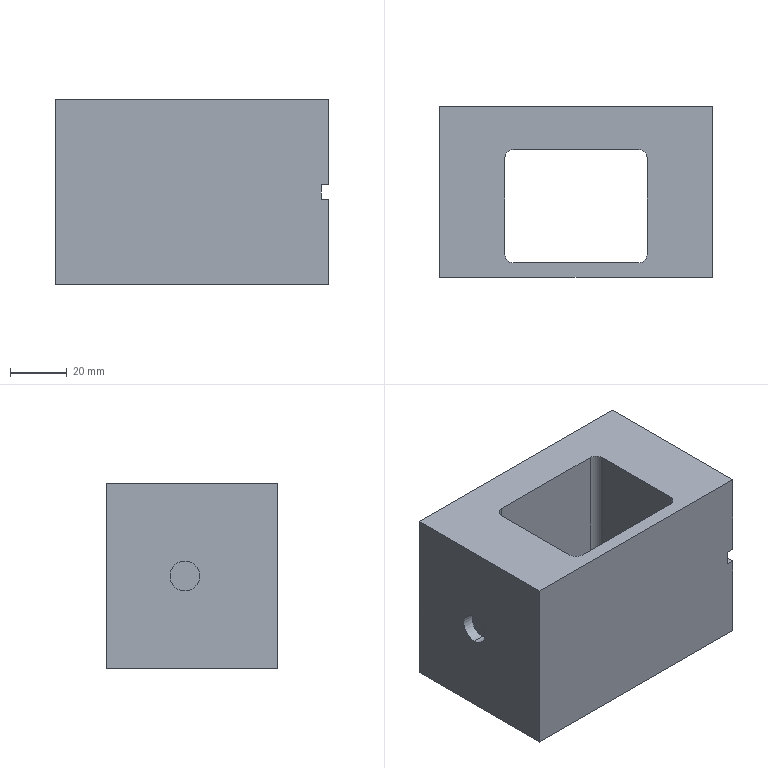Component | SolidWorks | CuttingDie-1_-Mold01-2-1 | 1 solid | 21 faces | box 96 x 60 x 65 mm | volume 243806 mm3 | plane 15 | cylinder 6 | commonest cylinder face diameters 6 x4 10.5 x2
build123d program:
from build123d import *

# Parameters (mm, degrees)
SKETCH1_W           = 65
SKETCH1_H           = 96
BOSS_EXTRUDE1_DEPTH = 32.5
SKETCH3_W           = 5
SKETCH3_H           = 2.5
CUT_EXTRUDE2_DEPTH  = 88.093
SKETCH4_R           = 5.25
CUT_EXTRUDE3_DEPTH  = 4
SKETCH6_W           = 65
SKETCH6_H           = 5
CUT_EXTRUDE5_DEPTH  = 107.435
CUT_EXTRUDE7_DEPTH  = 88.093


with BuildPart() as part:
    # Sketch1 → Boss-Extrude1 (new, symmetric)
    with BuildSketch(Plane(origin=(0, 0, 0), x_dir=(1, 0, 0), z_dir=(0, 1, 0))):
        Rectangle(SKETCH1_W, SKETCH1_H)
    extrude(amount=BOSS_EXTRUDE1_DEPTH, both=True)

    # Sketch3 → Cut-Extrude2 (cut, through all)
    with BuildSketch(Plane(origin=(0, 32.5, 0), x_dir=(1, 0, 0), z_dir=(0, 1, 0))):
        with Locations((0, 46.75)):
            Rectangle(SKETCH3_W, SKETCH3_H)
    extrude(amount=-CUT_EXTRUDE2_DEPTH, mode=Mode.SUBTRACT)

    # Sketch4 → Cut-Extrude3 (cut)
    with BuildSketch(Plane.XY.offset(48)):
        Circle(SKETCH4_R)
    extrude(amount=-CUT_EXTRUDE3_DEPTH, mode=Mode.SUBTRACT)

    # Sketch6 → Cut-Extrude5 (cut, through all)
    with BuildSketch(Plane.XY.offset(48)):
        with Locations((0, 30)):
            Rectangle(SKETCH6_W, SKETCH6_H)
    extrude(amount=-CUT_EXTRUDE5_DEPTH, mode=Mode.SUBTRACT)

    # Sketch2 → Cut-Extrude7 (cut, through all)
    with BuildSketch(Plane(origin=(32.5, 0, 0), x_dir=(0, 0, -1), z_dir=(1, 0, 0))):
        with BuildLine():
            Line((-22, -27.5), (22, -27.5))
            ThreePointArc((22, -27.5), (24.121, -26.621), (25, -24.5))
            Line((25, -24.5), (25, 9.5))
            ThreePointArc((25, 9.5), (24.121, 11.621), (22, 12.5))
            Line((22, 12.5), (-22, 12.5))
            ThreePointArc((-22, 12.5), (-24.121, 11.621), (-25, 9.5))
            Line((-25, 9.5), (-25, -24.5))
            ThreePointArc((-25, -24.5), (-24.121, -26.621), (-22, -27.5))
        make_face()
    extrude(amount=-CUT_EXTRUDE7_DEPTH, mode=Mode.SUBTRACT)


solid = part.part

# Placed as in the assembly
solid = solid.moved(Location((-439.272, -274.266, 1034.5), (0, -90, 0)))
STEP:
#1=COLOUR_RGB('',0.7922,0.8196,0.9333);
#2=FILL_AREA_STYLE_COLOUR('',#1);
#3=FILL_AREA_STYLE('',(#2));
#4=SURFACE_STYLE_FILL_AREA(#3);
#5=SURFACE_SIDE_STYLE('',(#4));
#6=SURFACE_STYLE_USAGE(.BOTH.,#5);
#7=PRESENTATION_STYLE_ASSIGNMENT((#6));
#8=CARTESIAN_POINT('',(-19.026,-10.798,40.522));
#9=VERTEX_POINT('',#8);
#10=CARTESIAN_POINT('',(-19.026,-10.798,40.935));
#11=VERTEX_POINT('',#10);
#12=CARTESIAN_POINT('',(-19.026,-10.798,40.728));
#13=DIRECTION('',(-1.,-0.,-0.));
#14=DIRECTION('',(0.,0.,1.));
#15=AXIS2_PLACEMENT_3D('',#12,#13,#14);
#16=CIRCLE('',#15,0.2067);
#17=EDGE_CURVE('',#9,#11,#16,.T.);
#18=ORIENTED_EDGE('',*,*,#17,.F.);
#19=CARTESIAN_POINT('',(-19.184,-10.798,40.522));
#20=VERTEX_POINT('',#19);
#21=CARTESIAN_POINT('',(-19.026,-10.798,40.522));
#22=DIRECTION('',(-1.,-0.,-0.));
#23=VECTOR('',#22,39.37);
#24=LINE('',#21,#23);
#25=EDGE_CURVE('',#9,#20,#24,.T.);
#26=ORIENTED_EDGE('',*,*,#25,.T.);
#27=CARTESIAN_POINT('',(-19.184,-10.798,40.935));
#28=VERTEX_POINT('',#27);
#29=CARTESIAN_POINT('',(-19.184,-10.798,40.728));
#30=DIRECTION('',(-1.,-0.,-0.));
#31=DIRECTION('',(0.,0.,1.));
#32=AXIS2_PLACEMENT_3D('',#29,#30,#31);
#33=CIRCLE('',#32,0.2067);
#34=EDGE_CURVE('',#20,#28,#33,.T.);
#35=ORIENTED_EDGE('',*,*,#34,.T.);
#36=CARTESIAN_POINT('',(-19.026,-10.798,40.935));
#37=DIRECTION('',(-1.,-0.,-0.));
#38=VECTOR('',#37,39.37);
#39=LINE('',#36,#38);
#40=EDGE_CURVE('',#11,#28,#39,.T.);
#41=ORIENTED_EDGE('',*,*,#40,.F.);
#42=EDGE_LOOP('',(#18,#26,#35,#41));
#43=FACE_OUTER_BOUND('',#42,.T.);
#44=CARTESIAN_POINT('',(-19.026,-10.798,40.728));
#45=DIRECTION('',(-1.,-0.,-0.));
#46=DIRECTION('',(0.,0.,1.));
#47=AXIS2_PLACEMENT_3D('',#44,#45,#46);
#48=CYLINDRICAL_SURFACE('',#47,0.2067);
#49=ADVANCED_FACE('',(#43),#48,.F.);
#50=CARTESIAN_POINT('',(-15.404,-9.715,39.449));
#51=VERTEX_POINT('',#50);
#52=CARTESIAN_POINT('',(-15.404,-12.077,39.449));
#53=VERTEX_POINT('',#52);
#54=CARTESIAN_POINT('',(-15.404,-9.518,39.449));
#55=DIRECTION('',(0.,-1.,-0.));
#56=VECTOR('',#55,39.37);
#57=LINE('',#54,#56);
#58=EDGE_CURVE('',#51,#53,#57,.T.);
#59=ORIENTED_EDGE('',*,*,#58,.F.);
#60=CARTESIAN_POINT('',(-15.404,-9.715,40.63));
#61=VERTEX_POINT('',#60);
#62=CARTESIAN_POINT('',(-15.404,-9.715,39.449));
#63=DIRECTION('',(-0.,-0.,1.));
#64=VECTOR('',#63,39.37);
#65=LINE('',#62,#64);
#66=EDGE_CURVE('',#51,#61,#65,.T.);
#67=ORIENTED_EDGE('',*,*,#66,.T.);
#68=CARTESIAN_POINT('',(-15.404,-12.077,40.63));
#69=VERTEX_POINT('',#68);
#70=CARTESIAN_POINT('',(-15.404,-12.077,40.63));
#71=DIRECTION('',(-0.,1.,0.));
#72=VECTOR('',#71,39.37);
#73=LINE('',#70,#72);
#74=EDGE_CURVE('',#69,#61,#73,.T.);
#75=ORIENTED_EDGE('',*,*,#74,.F.);
#76=CARTESIAN_POINT('',(-15.404,-12.077,39.449));
#77=DIRECTION('',(0.,0.,-1.));
#78=VECTOR('',#77,39.37);
#79=LINE('',#76,#78);
#80=EDGE_CURVE('',#69,#53,#79,.T.);
#81=ORIENTED_EDGE('',*,*,#80,.T.);
#82=EDGE_LOOP('',(#59,#67,#75,#81));
#83=FACE_OUTER_BOUND('',#82,.T.);
#84=CARTESIAN_POINT('',(-15.404,-9.518,39.449));
#85=DIRECTION('',(-1.,-0.,-0.));
#86=DIRECTION('',(-0.,-0.,1.));
#87=AXIS2_PLACEMENT_3D('',#84,#85,#86);
#88=PLANE('',#87);
#89=ADVANCED_FACE('',(#83),#88,.F.);
#90=CARTESIAN_POINT('',(-16.31,-11.762,42.008));
#91=VERTEX_POINT('',#90);
#92=CARTESIAN_POINT('',(-16.31,-10.424,42.008));
#93=VERTEX_POINT('',#92);
#94=CARTESIAN_POINT('',(-16.31,-11.762,42.008));
#95=DIRECTION('',(-0.,1.,0.));
#96=VECTOR('',#95,39.37);
#97=LINE('',#94,#96);
#98=EDGE_CURVE('',#91,#93,#97,.T.);
#99=ORIENTED_EDGE('',*,*,#98,.F.);
#100=CARTESIAN_POINT('',(-16.428,-11.881,42.008));
#101=VERTEX_POINT('',#100);
#102=CARTESIAN_POINT('',(-16.428,-11.762,42.008));
#103=DIRECTION('',(-0.,-0.,1.));
#104=DIRECTION('',(1.,0.,0.));
#105=AXIS2_PLACEMENT_3D('',#102,#103,#104);
#106=CIRCLE('',#105,0.1181);
#107=EDGE_CURVE('',#101,#91,#106,.T.);
#108=ORIENTED_EDGE('',*,*,#107,.F.);
#109=CARTESIAN_POINT('',(-18.16,-11.881,42.008));
#110=VERTEX_POINT('',#109);
#111=CARTESIAN_POINT('',(-18.16,-11.881,42.008));
#112=DIRECTION('',(1.,0.,0.));
#113=VECTOR('',#112,39.37);
#114=LINE('',#111,#113);
#115=EDGE_CURVE('',#110,#101,#114,.T.);
#116=ORIENTED_EDGE('',*,*,#115,.F.);
#117=CARTESIAN_POINT('',(-18.278,-11.762,42.008));
#118=VERTEX_POINT('',#117);
#119=CARTESIAN_POINT('',(-18.16,-11.762,42.008));
#120=DIRECTION('',(-0.,-0.,1.));
#121=DIRECTION('',(-1.,0.,0.));
#122=AXIS2_PLACEMENT_3D('',#119,#120,#121);
#123=CIRCLE('',#122,0.1181);
#124=EDGE_CURVE('',#118,#110,#123,.T.);
#125=ORIENTED_EDGE('',*,*,#124,.F.);
#126=CARTESIAN_POINT('',(-18.278,-10.424,42.008));
#127=VERTEX_POINT('',#126);
#128=CARTESIAN_POINT('',(-18.278,-11.762,42.008));
#129=DIRECTION('',(0.,-1.,-0.));
#130=VECTOR('',#129,39.37);
#131=LINE('',#128,#130);
#132=EDGE_CURVE('',#127,#118,#131,.T.);
#133=ORIENTED_EDGE('',*,*,#132,.F.);
#134=CARTESIAN_POINT('',(-18.16,-10.306,42.008));
#135=VERTEX_POINT('',#134);
#136=CARTESIAN_POINT('',(-18.16,-10.424,42.008));
#137=DIRECTION('',(-0.,-0.,1.));
#138=DIRECTION('',(-1.,0.,0.));
#139=AXIS2_PLACEMENT_3D('',#136,#137,#138);
#140=CIRCLE('',#139,0.1181);
#141=EDGE_CURVE('',#135,#127,#140,.T.);
#142=ORIENTED_EDGE('',*,*,#141,.F.);
#143=CARTESIAN_POINT('',(-16.428,-10.306,42.008));
#144=VERTEX_POINT('',#143);
#145=CARTESIAN_POINT('',(-18.16,-10.306,42.008));
#146=DIRECTION('',(-1.,-0.,-0.));
#147=VECTOR('',#146,39.37);
#148=LINE('',#145,#147);
#149=EDGE_CURVE('',#144,#135,#148,.T.);
#150=ORIENTED_EDGE('',*,*,#149,.F.);
#151=CARTESIAN_POINT('',(-16.428,-10.424,42.008));
#152=DIRECTION('',(-0.,-0.,1.));
#153=DIRECTION('',(-1.,0.,0.));
#154=AXIS2_PLACEMENT_3D('',#151,#152,#153);
#155=CIRCLE('',#154,0.1181);
#156=EDGE_CURVE('',#93,#144,#155,.T.);
#157=ORIENTED_EDGE('',*,*,#156,.F.);
#158=EDGE_LOOP('',(#99,#108,#116,#125,#133,#142,#150,#157));
#159=FACE_BOUND('',#158,.T.);
#160=CARTESIAN_POINT('',(-15.404,-9.715,42.008));
#161=VERTEX_POINT('',#160);
#162=CARTESIAN_POINT('',(-15.404,-12.077,42.008));
#163=VERTEX_POINT('',#162);
#164=CARTESIAN_POINT('',(-15.404,-9.518,42.008));
#165=DIRECTION('',(0.,-1.,-0.));
#166=VECTOR('',#165,39.37);
#167=LINE('',#164,#166);
#168=EDGE_CURVE('',#161,#163,#167,.T.);
#169=ORIENTED_EDGE('',*,*,#168,.F.);
#170=CARTESIAN_POINT('',(-19.184,-9.715,42.008));
#171=VERTEX_POINT('',#170);
#172=CARTESIAN_POINT('',(-15.404,-9.715,42.008));
#173=DIRECTION('',(-1.,-0.,-0.));
#174=VECTOR('',#173,39.37);
#175=LINE('',#172,#174);
#176=EDGE_CURVE('',#161,#171,#175,.T.);
#177=ORIENTED_EDGE('',*,*,#176,.T.);
#178=CARTESIAN_POINT('',(-19.184,-12.077,42.008));
#179=VERTEX_POINT('',#178);
#180=CARTESIAN_POINT('',(-19.184,-9.518,42.008));
#181=DIRECTION('',(0.,-1.,-0.));
#182=VECTOR('',#181,39.37);
#183=LINE('',#180,#182);
#184=EDGE_CURVE('',#171,#179,#183,.T.);
#185=ORIENTED_EDGE('',*,*,#184,.T.);
#186=CARTESIAN_POINT('',(-19.184,-12.077,42.008));
#187=DIRECTION('',(1.,0.,0.));
#188=VECTOR('',#187,39.37);
#189=LINE('',#186,#188);
#190=EDGE_CURVE('',#179,#163,#189,.T.);
#191=ORIENTED_EDGE('',*,*,#190,.T.);
#192=EDGE_LOOP('',(#169,#177,#185,#191));
#193=FACE_OUTER_BOUND('',#192,.T.);
#194=CARTESIAN_POINT('',(-19.184,-9.518,42.008));
#195=DIRECTION('',(0.,0.,-1.));
#196=DIRECTION('',(-1.,-0.,-0.));
#197=AXIS2_PLACEMENT_3D('',#194,#195,#196);
#198=PLANE('',#197);
#199=ADVANCED_FACE('',(#159,#193),#198,.F.);
#200=CARTESIAN_POINT('',(-15.404,-12.077,40.827));
#201=VERTEX_POINT('',#200);
#202=CARTESIAN_POINT('',(-15.404,-9.715,40.827));
#203=VERTEX_POINT('',#202);
#204=CARTESIAN_POINT('',(-15.404,-12.077,40.827));
#205=DIRECTION('',(-0.,1.,0.));
#206=VECTOR('',#205,39.37);
#207=LINE('',#204,#206);
#208=EDGE_CURVE('',#201,#203,#207,.T.);
#209=ORIENTED_EDGE('',*,*,#208,.T.);
#210=CARTESIAN_POINT('',(-15.404,-9.715,39.449));
#211=DIRECTION('',(-0.,-0.,1.));
#212=VECTOR('',#211,39.37);
#213=LINE('',#210,#212);
#214=EDGE_CURVE('',#203,#161,#213,.T.);
#215=ORIENTED_EDGE('',*,*,#214,.T.);
#216=ORIENTED_EDGE('',*,*,#168,.T.);
#217=CARTESIAN_POINT('',(-15.404,-12.077,39.449));
#218=DIRECTION('',(0.,0.,-1.));
#219=VECTOR('',#218,39.37);
#220=LINE('',#217,#219);
#221=EDGE_CURVE('',#163,#201,#220,.T.);
#222=ORIENTED_EDGE('',*,*,#221,.T.);
#223=EDGE_LOOP('',(#209,#215,#216,#222));
#224=FACE_OUTER_BOUND('',#223,.T.);
#225=CARTESIAN_POINT('',(-15.404,-9.518,39.449));
#226=DIRECTION('',(-1.,-0.,-0.));
#227=DIRECTION('',(-0.,-0.,1.));
#228=AXIS2_PLACEMENT_3D('',#225,#226,#227);
#229=PLANE('',#228);
#230=ADVANCED_FACE('',(#224),#229,.F.);
#231=CARTESIAN_POINT('',(-18.16,-11.881,39.449));
#232=VERTEX_POINT('',#231);
#233=CARTESIAN_POINT('',(-16.428,-11.881,39.449));
#234=VERTEX_POINT('',#233);
#235=CARTESIAN_POINT('',(-18.16,-11.881,39.449));
#236=DIRECTION('',(1.,0.,0.));
#237=VECTOR('',#236,39.37);
#238=LINE('',#235,#237);
#239=EDGE_CURVE('',#232,#234,#238,.T.);
#240=ORIENTED_EDGE('',*,*,#239,.T.);
#241=CARTESIAN_POINT('',(-16.31,-11.762,39.449));
#242=VERTEX_POINT('',#241);
#243=CARTESIAN_POINT('',(-16.428,-11.762,39.449));
#244=DIRECTION('',(-0.,-0.,1.));
#245=DIRECTION('',(1.,0.,0.));
#246=AXIS2_PLACEMENT_3D('',#243,#244,#245);
#247=CIRCLE('',#246,0.1181);
#248=EDGE_CURVE('',#234,#242,#247,.T.);
#249=ORIENTED_EDGE('',*,*,#248,.T.);
#250=CARTESIAN_POINT('',(-16.31,-10.424,39.449));
#251=VERTEX_POINT('',#250);
#252=CARTESIAN_POINT('',(-16.31,-11.762,39.449));
#253=DIRECTION('',(-0.,1.,0.));
#254=VECTOR('',#253,39.37);
#255=LINE('',#252,#254);
#256=EDGE_CURVE('',#242,#251,#255,.T.);
#257=ORIENTED_EDGE('',*,*,#256,.T.);
#258=CARTESIAN_POINT('',(-16.428,-10.306,39.449));
#259=VERTEX_POINT('',#258);
#260=CARTESIAN_POINT('',(-16.428,-10.424,39.449));
#261=DIRECTION('',(-0.,-0.,1.));
#262=DIRECTION('',(-1.,0.,0.));
#263=AXIS2_PLACEMENT_3D('',#260,#261,#262);
#264=CIRCLE('',#263,0.1181);
#265=EDGE_CURVE('',#251,#259,#264,.T.);
#266=ORIENTED_EDGE('',*,*,#265,.T.);
#267=CARTESIAN_POINT('',(-18.16,-10.306,39.449));
#268=VERTEX_POINT('',#267);
#269=CARTESIAN_POINT('',(-18.16,-10.306,39.449));
#270=DIRECTION('',(-1.,-0.,-0.));
#271=VECTOR('',#270,39.37);
#272=LINE('',#269,#271);
#273=EDGE_CURVE('',#259,#268,#272,.T.);
#274=ORIENTED_EDGE('',*,*,#273,.T.);
#275=CARTESIAN_POINT('',(-18.278,-10.424,39.449));
#276=VERTEX_POINT('',#275);
#277=CARTESIAN_POINT('',(-18.16,-10.424,39.449));
#278=DIRECTION('',(-0.,-0.,1.));
#279=DIRECTION('',(-1.,0.,0.));
#280=AXIS2_PLACEMENT_3D('',#277,#278,#279);
#281=CIRCLE('',#280,0.1181);
#282=EDGE_CURVE('',#268,#276,#281,.T.);
#283=ORIENTED_EDGE('',*,*,#282,.T.);
#284=CARTESIAN_POINT('',(-18.278,-11.762,39.449));
#285=VERTEX_POINT('',#284);
#286=CARTESIAN_POINT('',(-18.278,-11.762,39.449));
#287=DIRECTION('',(0.,-1.,-0.));
#288=VECTOR('',#287,39.37);
#289=LINE('',#286,#288);
#290=EDGE_CURVE('',#276,#285,#289,.T.);
#291=ORIENTED_EDGE('',*,*,#290,.T.);
#292=CARTESIAN_POINT('',(-18.16,-11.762,39.449));
#293=DIRECTION('',(-0.,-0.,1.));
#294=DIRECTION('',(-1.,0.,0.));
#295=AXIS2_PLACEMENT_3D('',#292,#293,#294);
#296=CIRCLE('',#295,0.1181);
#297=EDGE_CURVE('',#285,#232,#296,.T.);
#298=ORIENTED_EDGE('',*,*,#297,.T.);
#299=EDGE_LOOP('',(#240,#249,#257,#266,#274,#283,#291,#298));
#300=FACE_BOUND('',#299,.T.);
#301=CARTESIAN_POINT('',(-19.184,-9.715,39.449));
#302=VERTEX_POINT('',#301);
#303=CARTESIAN_POINT('',(-19.184,-12.077,39.449));
#304=VERTEX_POINT('',#303);
#305=CARTESIAN_POINT('',(-19.184,-9.518,39.449));
#306=DIRECTION('',(0.,-1.,-0.));
#307=VECTOR('',#306,39.37);
#308=LINE('',#305,#307);
#309=EDGE_CURVE('',#302,#304,#308,.T.);
#310=ORIENTED_EDGE('',*,*,#309,.F.);
#311=CARTESIAN_POINT('',(-15.404,-9.715,39.449));
#312=DIRECTION('',(-1.,-0.,-0.));
#313=VECTOR('',#312,39.37);
#314=LINE('',#311,#313);
#315=EDGE_CURVE('',#51,#302,#314,.T.);
#316=ORIENTED_EDGE('',*,*,#315,.F.);
#317=ORIENTED_EDGE('',*,*,#58,.T.);
#318=CARTESIAN_POINT('',(-19.184,-12.077,39.449));
#319=DIRECTION('',(-1.,-0.,-0.));
#320=VECTOR('',#319,39.37);
#321=LINE('',#318,#320);
#322=EDGE_CURVE('',#53,#304,#321,.T.);
#323=ORIENTED_EDGE('',*,*,#322,.T.);
#324=EDGE_LOOP('',(#310,#316,#317,#323));
#325=FACE_OUTER_BOUND('',#324,.T.);
#326=CARTESIAN_POINT('',(-19.184,-9.518,39.449));
#327=DIRECTION('',(-0.,-0.,1.));
#328=DIRECTION('',(1.,0.,0.));
#329=AXIS2_PLACEMENT_3D('',#326,#327,#328);
#330=PLANE('',#329);
#331=ADVANCED_FACE('',(#300,#325),#330,.F.);
#332=CARTESIAN_POINT('',(-19.184,-10.798,40.728));
#333=DIRECTION('',(-1.,-0.,-0.));
#334=DIRECTION('',(0.,0.,1.));
#335=AXIS2_PLACEMENT_3D('',#332,#333,#334);
#336=CIRCLE('',#335,0.2067);
#337=EDGE_CURVE('',#28,#20,#336,.T.);
#338=ORIENTED_EDGE('',*,*,#337,.F.);
#339=ORIENTED_EDGE('',*,*,#34,.F.);
#340=EDGE_LOOP('',(#338,#339));
#341=FACE_BOUND('',#340,.T.);
#342=ORIENTED_EDGE('',*,*,#184,.F.);
#343=CARTESIAN_POINT('',(-19.184,-9.715,39.449));
#344=DIRECTION('',(-0.,-0.,1.));
#345=VECTOR('',#344,39.37);
#346=LINE('',#343,#345);
#347=EDGE_CURVE('',#302,#171,#346,.T.);
#348=ORIENTED_EDGE('',*,*,#347,.F.);
#349=ORIENTED_EDGE('',*,*,#309,.T.);
#350=CARTESIAN_POINT('',(-19.184,-12.077,39.449));
#351=DIRECTION('',(-0.,-0.,1.));
#352=VECTOR('',#351,39.37);
#353=LINE('',#350,#352);
#354=EDGE_CURVE('',#304,#179,#353,.T.);
#355=ORIENTED_EDGE('',*,*,#354,.T.);
#356=EDGE_LOOP('',(#342,#348,#349,#355));
#357=FACE_OUTER_BOUND('',#356,.T.);
#358=CARTESIAN_POINT('',(-19.184,-9.518,39.449));
#359=DIRECTION('',(1.,0.,0.));
#360=DIRECTION('',(0.,0.,-1.));
#361=AXIS2_PLACEMENT_3D('',#358,#359,#360);
#362=PLANE('',#361);
#363=ADVANCED_FACE('',(#341,#357),#362,.F.);
#364=CARTESIAN_POINT('',(-15.503,-12.077,40.63));
#365=VERTEX_POINT('',#364);
#366=CARTESIAN_POINT('',(-15.404,-12.077,40.63));
#367=DIRECTION('',(-1.,-0.,-0.));
#368=VECTOR('',#367,39.37);
#369=LINE('',#366,#368);
#370=EDGE_CURVE('',#69,#365,#369,.T.);
#371=ORIENTED_EDGE('',*,*,#370,.T.);
#372=CARTESIAN_POINT('',(-15.503,-12.077,40.827));
#373=VERTEX_POINT('',#372);
#374=CARTESIAN_POINT('',(-15.503,-12.077,40.63));
#375=DIRECTION('',(-0.,-0.,1.));
#376=VECTOR('',#375,39.37);
#377=LINE('',#374,#376);
#378=EDGE_CURVE('',#365,#373,#377,.T.);
#379=ORIENTED_EDGE('',*,*,#378,.T.);
#380=CARTESIAN_POINT('',(-15.404,-12.077,40.827));
#381=DIRECTION('',(1.,0.,0.));
#382=VECTOR('',#381,39.37);
#383=LINE('',#380,#382);
#384=EDGE_CURVE('',#373,#201,#383,.T.);
#385=ORIENTED_EDGE('',*,*,#384,.T.);
#386=ORIENTED_EDGE('',*,*,#221,.F.);
#387=ORIENTED_EDGE('',*,*,#190,.F.);
#388=ORIENTED_EDGE('',*,*,#354,.F.);
#389=ORIENTED_EDGE('',*,*,#322,.F.);
#390=ORIENTED_EDGE('',*,*,#80,.F.);
#391=EDGE_LOOP('',(#371,#379,#385,#386,#387,#388,#389,#390));
#392=FACE_OUTER_BOUND('',#391,.T.);
#393=CARTESIAN_POINT('',(-17.294,-12.077,40.728));
#394=DIRECTION('',(0.,-1.,-0.));
#395=DIRECTION('',(1.,0.,0.));
#396=AXIS2_PLACEMENT_3D('',#393,#394,#395);
#397=PLANE('',#396);
#398=ADVANCED_FACE('',(#392),#397,.T.);
#399=ORIENTED_EDGE('',*,*,#74,.T.);
#400=CARTESIAN_POINT('',(-15.503,-9.715,40.63));
#401=VERTEX_POINT('',#400);
#402=CARTESIAN_POINT('',(-15.404,-9.715,40.63));
#403=DIRECTION('',(-1.,-0.,-0.));
#404=VECTOR('',#403,39.37);
#405=LINE('',#402,#404);
#406=EDGE_CURVE('',#61,#401,#405,.T.);
#407=ORIENTED_EDGE('',*,*,#406,.T.);
#408=CARTESIAN_POINT('',(-15.503,-12.077,40.63));
#409=DIRECTION('',(-0.,1.,0.));
#410=VECTOR('',#409,39.37);
#411=LINE('',#408,#410);
#412=EDGE_CURVE('',#365,#401,#411,.T.);
#413=ORIENTED_EDGE('',*,*,#412,.F.);
#414=ORIENTED_EDGE('',*,*,#370,.F.);
#415=EDGE_LOOP('',(#399,#407,#413,#414));
#416=FACE_OUTER_BOUND('',#415,.T.);
#417=CARTESIAN_POINT('',(-15.404,-12.077,40.63));
#418=DIRECTION('',(0.,0.,-1.));
#419=DIRECTION('',(-1.,-0.,-0.));
#420=AXIS2_PLACEMENT_3D('',#417,#418,#419);
#421=PLANE('',#420);
#422=ADVANCED_FACE('',(#416),#421,.F.);
#423=CARTESIAN_POINT('',(-15.503,-9.715,40.827));
#424=VERTEX_POINT('',#423);
#425=CARTESIAN_POINT('',(-15.503,-12.077,40.827));
#426=DIRECTION('',(-0.,1.,0.));
#427=VECTOR('',#426,39.37);
#428=LINE('',#425,#427);
#429=EDGE_CURVE('',#373,#424,#428,.T.);
#430=ORIENTED_EDGE('',*,*,#429,.T.);
#431=CARTESIAN_POINT('',(-15.404,-9.715,40.827));
#432=DIRECTION('',(1.,0.,0.));
#433=VECTOR('',#432,39.37);
#434=LINE('',#431,#433);
#435=EDGE_CURVE('',#424,#203,#434,.T.);
#436=ORIENTED_EDGE('',*,*,#435,.T.);
#437=ORIENTED_EDGE('',*,*,#208,.F.);
#438=ORIENTED_EDGE('',*,*,#384,.F.);
#439=EDGE_LOOP('',(#430,#436,#437,#438));
#440=FACE_OUTER_BOUND('',#439,.T.);
#441=CARTESIAN_POINT('',(-15.404,-12.077,40.827));
#442=DIRECTION('',(-0.,-0.,1.));
#443=DIRECTION('',(1.,0.,0.));
#444=AXIS2_PLACEMENT_3D('',#441,#442,#443);
#445=PLANE('',#444);
#446=ADVANCED_FACE('',(#440),#445,.F.);
#447=ORIENTED_EDGE('',*,*,#412,.T.);
#448=CARTESIAN_POINT('',(-15.503,-9.715,40.63));
#449=DIRECTION('',(-0.,-0.,1.));
#450=VECTOR('',#449,39.37);
#451=LINE('',#448,#450);
#452=EDGE_CURVE('',#401,#424,#451,.T.);
#453=ORIENTED_EDGE('',*,*,#452,.T.);
#454=ORIENTED_EDGE('',*,*,#429,.F.);
#455=ORIENTED_EDGE('',*,*,#378,.F.);
#456=EDGE_LOOP('',(#447,#453,#454,#455));
#457=FACE_OUTER_BOUND('',#456,.T.);
#458=CARTESIAN_POINT('',(-15.503,-12.077,40.63));
#459=DIRECTION('',(-1.,-0.,-0.));
#460=DIRECTION('',(-0.,-0.,1.));
#461=AXIS2_PLACEMENT_3D('',#458,#459,#460);
#462=PLANE('',#461);
#463=ADVANCED_FACE('',(#457),#462,.F.);
#464=ORIENTED_EDGE('',*,*,#25,.F.);
#465=CARTESIAN_POINT('',(-19.026,-10.798,40.728));
#466=DIRECTION('',(-1.,-0.,-0.));
#467=DIRECTION('',(0.,0.,1.));
#468=AXIS2_PLACEMENT_3D('',#465,#466,#467);
#469=CIRCLE('',#468,0.2067);
#470=EDGE_CURVE('',#11,#9,#469,.T.);
#471=ORIENTED_EDGE('',*,*,#470,.F.);
#472=ORIENTED_EDGE('',*,*,#40,.T.);
#473=ORIENTED_EDGE('',*,*,#337,.T.);
#474=EDGE_LOOP('',(#464,#471,#472,#473));
#475=FACE_OUTER_BOUND('',#474,.T.);
#476=CARTESIAN_POINT('',(-19.026,-10.798,40.728));
#477=DIRECTION('',(-1.,-0.,-0.));
#478=DIRECTION('',(0.,0.,1.));
#479=AXIS2_PLACEMENT_3D('',#476,#477,#478);
#480=CYLINDRICAL_SURFACE('',#479,0.2067);
#481=ADVANCED_FACE('',(#475),#480,.F.);
#482=ORIENTED_EDGE('',*,*,#470,.T.);
#483=ORIENTED_EDGE('',*,*,#17,.T.);
#484=EDGE_LOOP('',(#482,#483));
#485=FACE_OUTER_BOUND('',#484,.T.);
#486=CARTESIAN_POINT('',(-19.026,-10.798,40.728));
#487=DIRECTION('',(-1.,-0.,-0.));
#488=DIRECTION('',(-0.,-0.,1.));
#489=AXIS2_PLACEMENT_3D('',#486,#487,#488);
#490=PLANE('',#489);
#491=ADVANCED_FACE('',(#485),#490,.T.);
#492=ORIENTED_EDGE('',*,*,#66,.F.);
#493=ORIENTED_EDGE('',*,*,#315,.T.);
#494=ORIENTED_EDGE('',*,*,#347,.T.);
#495=ORIENTED_EDGE('',*,*,#176,.F.);
#496=ORIENTED_EDGE('',*,*,#214,.F.);
#497=ORIENTED_EDGE('',*,*,#435,.F.);
#498=ORIENTED_EDGE('',*,*,#452,.F.);
#499=ORIENTED_EDGE('',*,*,#406,.F.);
#500=EDGE_LOOP('',(#492,#493,#494,#495,#496,#497,#498,#499));
#501=FACE_OUTER_BOUND('',#500,.T.);
#502=CARTESIAN_POINT('',(-15.404,-9.715,39.449));
#503=DIRECTION('',(0.,-1.,-0.));
#504=DIRECTION('',(1.,0.,0.));
#505=AXIS2_PLACEMENT_3D('',#502,#503,#504);
#506=PLANE('',#505);
#507=ADVANCED_FACE('',(#501),#506,.F.);
#508=ORIENTED_EDGE('',*,*,#107,.T.);
#509=CARTESIAN_POINT('',(-16.31,-11.762,39.449));
#510=DIRECTION('',(-0.,-0.,1.));
#511=VECTOR('',#510,39.37);
#512=LINE('',#509,#511);
#513=EDGE_CURVE('',#242,#91,#512,.T.);
#514=ORIENTED_EDGE('',*,*,#513,.F.);
#515=ORIENTED_EDGE('',*,*,#248,.F.);
#516=CARTESIAN_POINT('',(-16.428,-11.881,39.449));
#517=DIRECTION('',(-0.,-0.,1.));
#518=VECTOR('',#517,39.37);
#519=LINE('',#516,#518);
#520=EDGE_CURVE('',#234,#101,#519,.T.);
#521=ORIENTED_EDGE('',*,*,#520,.T.);
#522=EDGE_LOOP('',(#508,#514,#515,#521));
#523=FACE_OUTER_BOUND('',#522,.T.);
#524=CARTESIAN_POINT('',(-16.428,-11.762,39.449));
#525=DIRECTION('',(-0.,-0.,1.));
#526=DIRECTION('',(1.,0.,0.));
#527=AXIS2_PLACEMENT_3D('',#524,#525,#526);
#528=CYLINDRICAL_SURFACE('',#527,0.1181);
#529=ADVANCED_FACE('',(#523),#528,.F.);
#530=ORIENTED_EDGE('',*,*,#115,.T.);
#531=ORIENTED_EDGE('',*,*,#520,.F.);
#532=ORIENTED_EDGE('',*,*,#239,.F.);
#533=CARTESIAN_POINT('',(-18.16,-11.881,39.449));
#534=DIRECTION('',(-0.,-0.,1.));
#535=VECTOR('',#534,39.37);
#536=LINE('',#533,#535);
#537=EDGE_CURVE('',#232,#110,#536,.T.);
#538=ORIENTED_EDGE('',*,*,#537,.T.);
#539=EDGE_LOOP('',(#530,#531,#532,#538));
#540=FACE_OUTER_BOUND('',#539,.T.);
#541=CARTESIAN_POINT('',(-18.16,-11.881,39.449));
#542=DIRECTION('',(0.,-1.,-0.));
#543=DIRECTION('',(1.,0.,0.));
#544=AXIS2_PLACEMENT_3D('',#541,#542,#543);
#545=PLANE('',#544);
#546=ADVANCED_FACE('',(#540),#545,.F.);
#547=ORIENTED_EDGE('',*,*,#124,.T.);
#548=ORIENTED_EDGE('',*,*,#537,.F.);
#549=ORIENTED_EDGE('',*,*,#297,.F.);
#550=CARTESIAN_POINT('',(-18.278,-11.762,39.449));
#551=DIRECTION('',(-0.,-0.,1.));
#552=VECTOR('',#551,39.37);
#553=LINE('',#550,#552);
#554=EDGE_CURVE('',#285,#118,#553,.T.);
#555=ORIENTED_EDGE('',*,*,#554,.T.);
#556=EDGE_LOOP('',(#547,#548,#549,#555));
#557=FACE_OUTER_BOUND('',#556,.T.);
#558=CARTESIAN_POINT('',(-18.16,-11.762,39.449));
#559=DIRECTION('',(-0.,-0.,1.));
#560=DIRECTION('',(1.,0.,0.));
#561=AXIS2_PLACEMENT_3D('',#558,#559,#560);
#562=CYLINDRICAL_SURFACE('',#561,0.1181);
#563=ADVANCED_FACE('',(#557),#562,.F.);
#564=ORIENTED_EDGE('',*,*,#132,.T.);
#565=ORIENTED_EDGE('',*,*,#554,.F.);
#566=ORIENTED_EDGE('',*,*,#290,.F.);
#567=CARTESIAN_POINT('',(-18.278,-10.424,39.449));
#568=DIRECTION('',(-0.,-0.,1.));
#569=VECTOR('',#568,39.37);
#570=LINE('',#567,#569);
#571=EDGE_CURVE('',#276,#127,#570,.T.);
#572=ORIENTED_EDGE('',*,*,#571,.T.);
#573=EDGE_LOOP('',(#564,#565,#566,#572));
#574=FACE_OUTER_BOUND('',#573,.T.);
#575=CARTESIAN_POINT('',(-18.278,-11.762,39.449));
#576=DIRECTION('',(-1.,-0.,-0.));
#577=DIRECTION('',(-0.,-0.,1.));
#578=AXIS2_PLACEMENT_3D('',#575,#576,#577);
#579=PLANE('',#578);
#580=ADVANCED_FACE('',(#574),#579,.F.);
#581=ORIENTED_EDGE('',*,*,#141,.T.);
#582=ORIENTED_EDGE('',*,*,#571,.F.);
#583=ORIENTED_EDGE('',*,*,#282,.F.);
#584=CARTESIAN_POINT('',(-18.16,-10.306,39.449));
#585=DIRECTION('',(-0.,-0.,1.));
#586=VECTOR('',#585,39.37);
#587=LINE('',#584,#586);
#588=EDGE_CURVE('',#268,#135,#587,.T.);
#589=ORIENTED_EDGE('',*,*,#588,.T.);
#590=EDGE_LOOP('',(#581,#582,#583,#589));
#591=FACE_OUTER_BOUND('',#590,.T.);
#592=CARTESIAN_POINT('',(-18.16,-10.424,39.449));
#593=DIRECTION('',(-0.,-0.,1.));
#594=DIRECTION('',(1.,0.,0.));
#595=AXIS2_PLACEMENT_3D('',#592,#593,#594);
#596=CYLINDRICAL_SURFACE('',#595,0.1181);
#597=ADVANCED_FACE('',(#591),#596,.F.);
#598=ORIENTED_EDGE('',*,*,#149,.T.);
#599=ORIENTED_EDGE('',*,*,#588,.F.);
#600=ORIENTED_EDGE('',*,*,#273,.F.);
#601=CARTESIAN_POINT('',(-16.428,-10.306,39.449));
#602=DIRECTION('',(-0.,-0.,1.));
#603=VECTOR('',#602,39.37);
#604=LINE('',#601,#603);
#605=EDGE_CURVE('',#259,#144,#604,.T.);
#606=ORIENTED_EDGE('',*,*,#605,.T.);
#607=EDGE_LOOP('',(#598,#599,#600,#606));
#608=FACE_OUTER_BOUND('',#607,.T.);
#609=CARTESIAN_POINT('',(-18.16,-10.306,39.449));
#610=DIRECTION('',(-0.,1.,0.));
#611=DIRECTION('',(-1.,-0.,-0.));
#612=AXIS2_PLACEMENT_3D('',#609,#610,#611);
#613=PLANE('',#612);
#614=ADVANCED_FACE('',(#608),#613,.F.);
#615=ORIENTED_EDGE('',*,*,#156,.T.);
#616=ORIENTED_EDGE('',*,*,#605,.F.);
#617=ORIENTED_EDGE('',*,*,#265,.F.);
#618=CARTESIAN_POINT('',(-16.31,-10.424,39.449));
#619=DIRECTION('',(-0.,-0.,1.));
#620=VECTOR('',#619,39.37);
#621=LINE('',#618,#620);
#622=EDGE_CURVE('',#251,#93,#621,.T.);
#623=ORIENTED_EDGE('',*,*,#622,.T.);
#624=EDGE_LOOP('',(#615,#616,#617,#623));
#625=FACE_OUTER_BOUND('',#624,.T.);
#626=CARTESIAN_POINT('',(-16.428,-10.424,39.449));
#627=DIRECTION('',(-0.,-0.,1.));
#628=DIRECTION('',(1.,0.,0.));
#629=AXIS2_PLACEMENT_3D('',#626,#627,#628);
#630=CYLINDRICAL_SURFACE('',#629,0.1181);
#631=ADVANCED_FACE('',(#625),#630,.F.);
#632=ORIENTED_EDGE('',*,*,#98,.T.);
#633=ORIENTED_EDGE('',*,*,#622,.F.);
#634=ORIENTED_EDGE('',*,*,#256,.F.);
#635=ORIENTED_EDGE('',*,*,#513,.T.);
#636=EDGE_LOOP('',(#632,#633,#634,#635));
#637=FACE_OUTER_BOUND('',#636,.T.);
#638=CARTESIAN_POINT('',(-16.31,-11.762,39.449));
#639=DIRECTION('',(1.,0.,0.));
#640=DIRECTION('',(-0.,1.,0.));
#641=AXIS2_PLACEMENT_3D('',#638,#639,#640);
#642=PLANE('',#641);
#643=ADVANCED_FACE('',(#637),#642,.F.);
#644=CLOSED_SHELL('',(#49,#89,#199,#230,#331,#363,#398,#422,#446,#463,#481,#491,#507,#529,#546,#563,#580,#597,#614,#631,#643));
#645=MANIFOLD_SOLID_BREP('',#644);
#646=STYLED_ITEM('',(#7),#645);
#647=PRESENTATION_LAYER_ASSIGNMENT('','',(#646));
#648=(LENGTH_UNIT()NAMED_UNIT(*)SI_UNIT($,.METRE.));
#649=LENGTH_MEASURE_WITH_UNIT(LENGTH_MEASURE(0.0254),#648);
#650=DIMENSIONAL_EXPONENTS(1.,0.,0.,0.,0.,0.,0.);
#651=(CONVERSION_BASED_UNIT('',#649)LENGTH_UNIT()NAMED_UNIT(#650));
#652=UNCERTAINTY_MEASURE_WITH_UNIT(LENGTH_MEASURE(0.00001),#651,'','');
#653=(NAMED_UNIT(*)PLANE_ANGLE_UNIT()SI_UNIT($,.RADIAN.));
#654=(NAMED_UNIT(*)SI_UNIT($,.STERADIAN.)SOLID_ANGLE_UNIT());
#655=(GEOMETRIC_REPRESENTATION_CONTEXT(3)GLOBAL_UNCERTAINTY_ASSIGNED_CONTEXT((#652))GLOBAL_UNIT_ASSIGNED_CONTEXT((#651,#653,#654))REPRESENTATION_CONTEXT('',''));
#656=MECHANICAL_DESIGN_GEOMETRIC_PRESENTATION_REPRESENTATION('',(#646),#655);
#657=CARTESIAN_POINT('',(0.,0.,0.));
#658=DIRECTION('',(0.,0.,1.));
#659=DIRECTION('',(1.,0.,0.));
#660=AXIS2_PLACEMENT_3D('',#657,#658,#659);
#661=(LENGTH_UNIT()NAMED_UNIT(*)SI_UNIT($,.METRE.));
#662=LENGTH_MEASURE_WITH_UNIT(LENGTH_MEASURE(0.0254),#661);
#663=DIMENSIONAL_EXPONENTS(1.,0.,0.,0.,0.,0.,0.);
#664=(CONVERSION_BASED_UNIT('',#662)LENGTH_UNIT()NAMED_UNIT(#663));
#665=UNCERTAINTY_MEASURE_WITH_UNIT(LENGTH_MEASURE(0.00001),#664,'','');
#666=(NAMED_UNIT(*)PLANE_ANGLE_UNIT()SI_UNIT($,.RADIAN.));
#667=(NAMED_UNIT(*)SI_UNIT($,.STERADIAN.)SOLID_ANGLE_UNIT());
#668=(GEOMETRIC_REPRESENTATION_CONTEXT(3)GLOBAL_UNCERTAINTY_ASSIGNED_CONTEXT((#665))GLOBAL_UNIT_ASSIGNED_CONTEXT((#664,#666,#667))REPRESENTATION_CONTEXT('',''));
#669=ADVANCED_BREP_SHAPE_REPRESENTATION('',(#645,#660),#668);